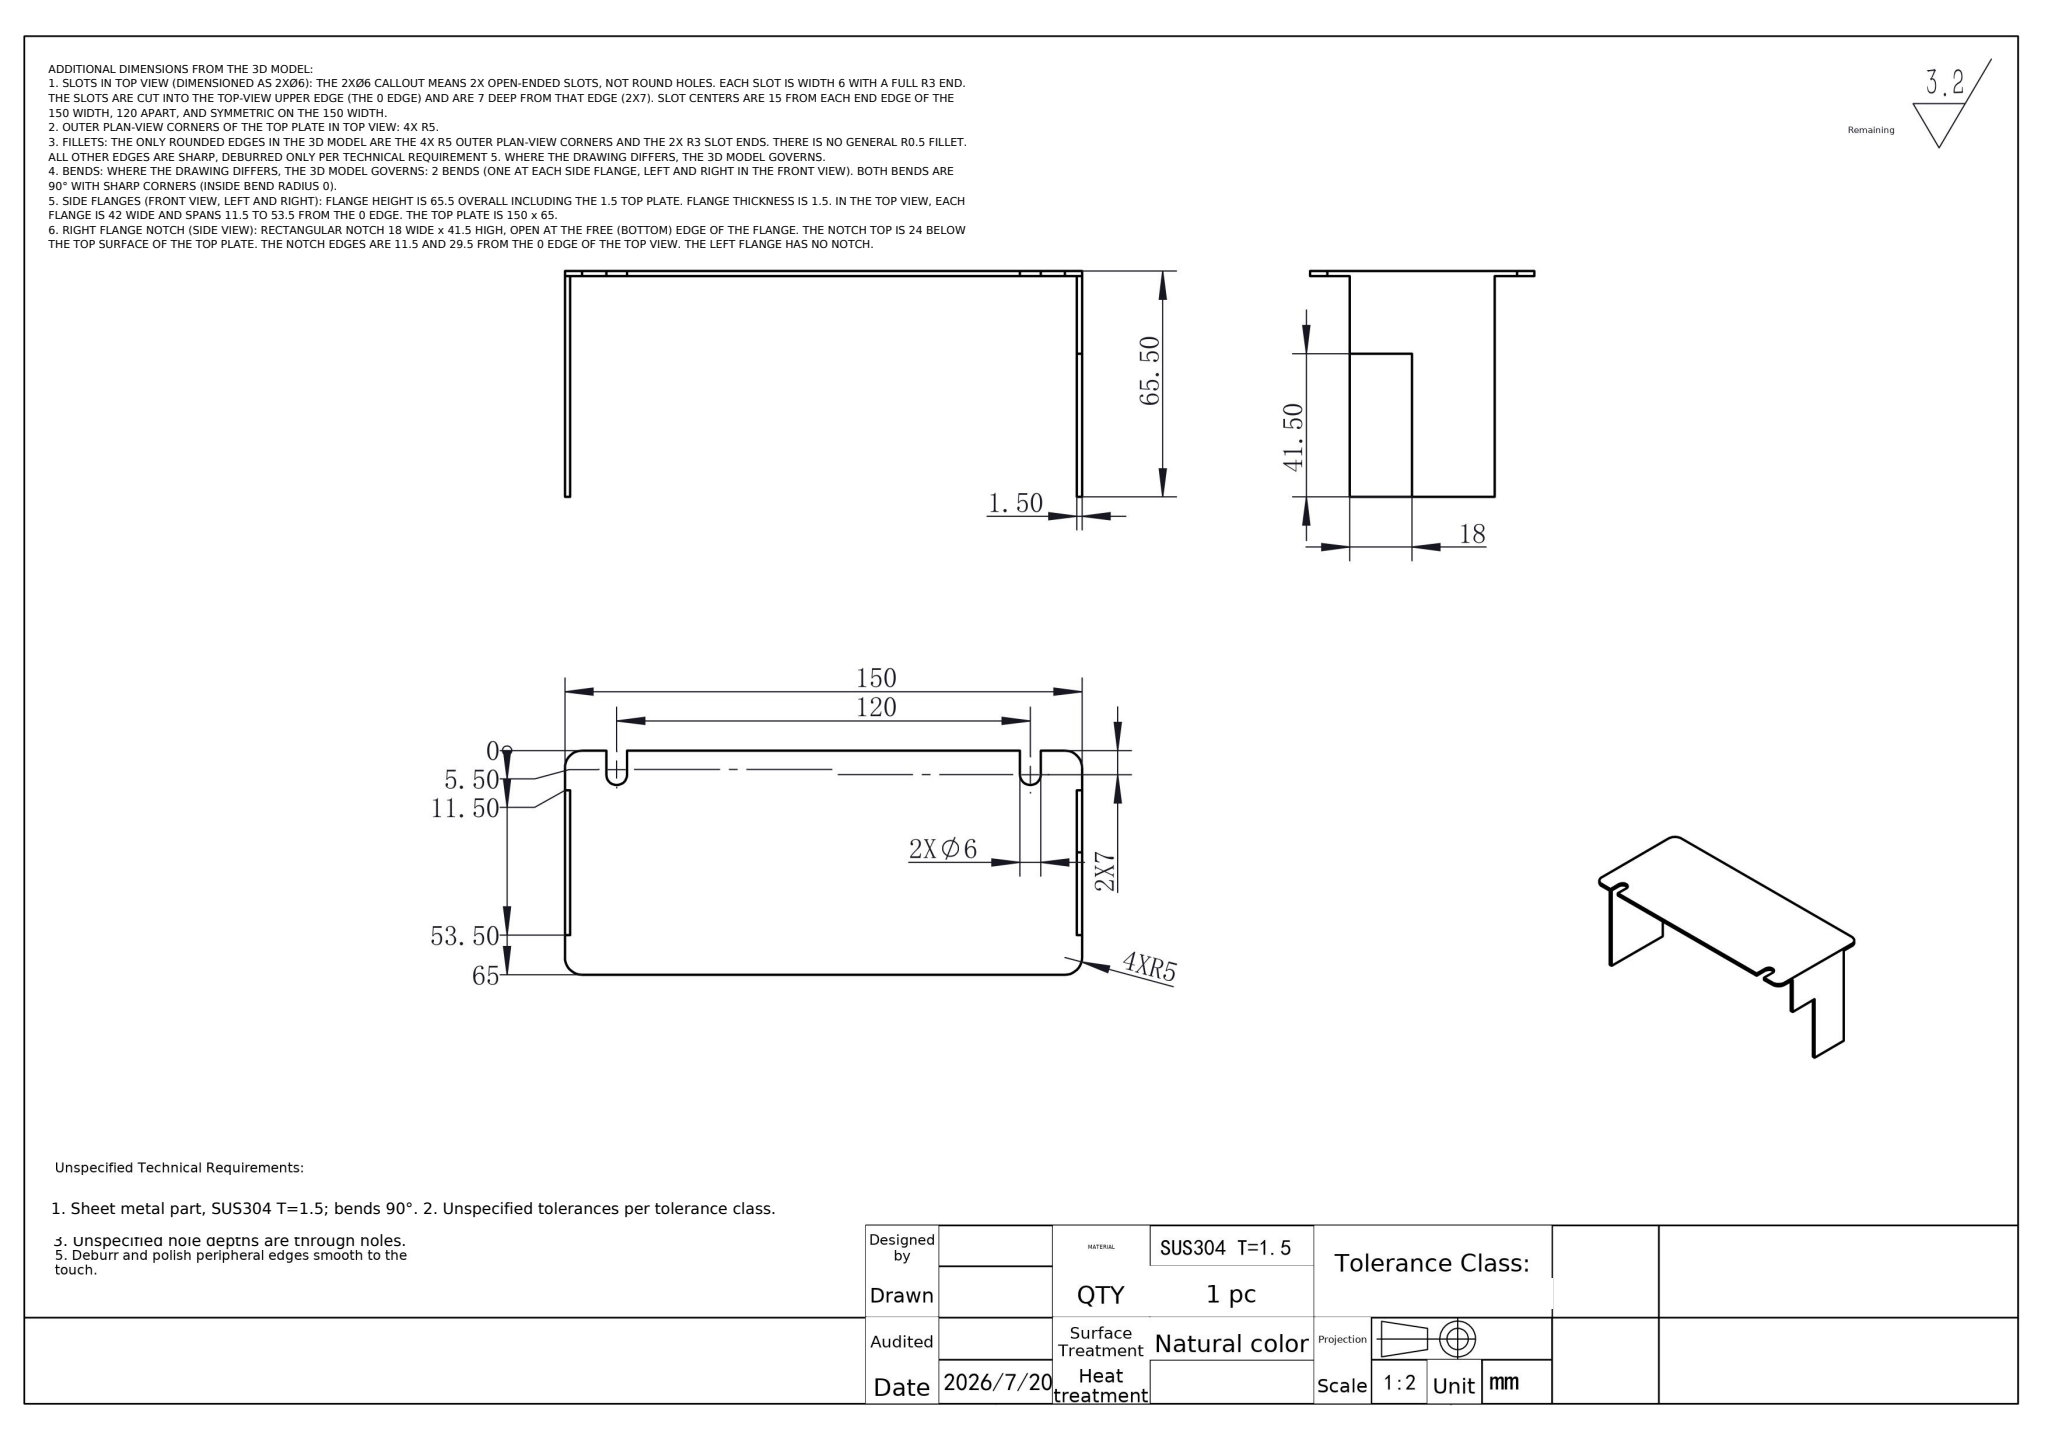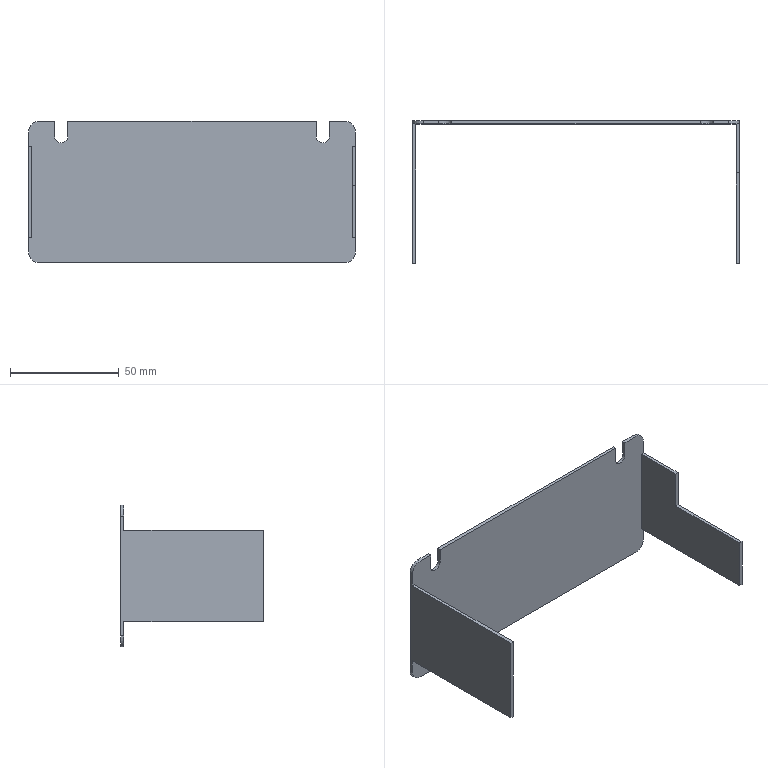Part | NX | mm | 1 solid | 28 faces | box 150 x 65.5 x 65 mm | volume 21368 mm3 | plane 22 | cylinder 6 | commonest cylinder face diameters 10 x4 6 x2
STEP:
#1=CARTESIAN_POINT('',(75.,0.,27.5));
#2=VERTEX_POINT('',#1);
#3=CARTESIAN_POINT('',(75.,0.,-27.5));
#4=VERTEX_POINT('',#3);
#5=CARTESIAN_POINT('',(75.,0.,32.5));
#6=DIRECTION('',(0.,0.,-1.));
#7=VECTOR('',#6,1000.);
#8=LINE('',#5,#7);
#9=EDGE_CURVE('',#2,#4,#8,.T.);
#10=ORIENTED_EDGE('',*,*,#9,.F.);
#11=CARTESIAN_POINT('',(75.,-1.5,27.5));
#12=VERTEX_POINT('',#11);
#13=CARTESIAN_POINT('',(75.,-1.5,27.5));
#14=DIRECTION('',(0.,-1.,0.));
#15=VECTOR('',#14,1000.);
#16=LINE('',#13,#15);
#17=EDGE_CURVE('',#2,#12,#16,.T.);
#18=ORIENTED_EDGE('',*,*,#17,.T.);
#19=CARTESIAN_POINT('',(75.,-1.5,21.));
#20=VERTEX_POINT('',#19);
#21=CARTESIAN_POINT('',(75.,-1.5,32.5));
#22=DIRECTION('',(0.,0.,-1.));
#23=VECTOR('',#22,1000.);
#24=LINE('',#21,#23);
#25=EDGE_CURVE('',#12,#20,#24,.T.);
#26=ORIENTED_EDGE('',*,*,#25,.T.);
#27=CARTESIAN_POINT('',(75.,-24.,21.));
#28=VERTEX_POINT('',#27);
#29=CARTESIAN_POINT('',(75.,-65.5,21.));
#30=DIRECTION('',(0.,1.,0.));
#31=VECTOR('',#30,1000.);
#32=LINE('',#29,#31);
#33=EDGE_CURVE('',#28,#20,#32,.T.);
#34=ORIENTED_EDGE('',*,*,#33,.F.);
#35=CARTESIAN_POINT('',(75.,-24.,3.));
#36=VERTEX_POINT('',#35);
#37=CARTESIAN_POINT('',(75.,-24.,3.));
#38=DIRECTION('',(0.,0.,-1.));
#39=VECTOR('',#38,1000.);
#40=LINE('',#37,#39);
#41=EDGE_CURVE('',#28,#36,#40,.T.);
#42=ORIENTED_EDGE('',*,*,#41,.T.);
#43=CARTESIAN_POINT('',(75.,-65.5,3.));
#44=VERTEX_POINT('',#43);
#45=CARTESIAN_POINT('',(75.,-100.5,3.));
#46=DIRECTION('',(0.,-1.,0.));
#47=VECTOR('',#46,1000.);
#48=LINE('',#45,#47);
#49=EDGE_CURVE('',#36,#44,#48,.T.);
#50=ORIENTED_EDGE('',*,*,#49,.T.);
#51=CARTESIAN_POINT('',(75.,-65.5,-21.));
#52=VERTEX_POINT('',#51);
#53=CARTESIAN_POINT('',(75.,-65.5,21.));
#54=DIRECTION('',(0.,0.,1.));
#55=VECTOR('',#54,1000.);
#56=LINE('',#53,#55);
#57=EDGE_CURVE('',#52,#44,#56,.T.);
#58=ORIENTED_EDGE('',*,*,#57,.F.);
#59=CARTESIAN_POINT('',(75.,-1.5,-21.));
#60=VERTEX_POINT('',#59);
#61=CARTESIAN_POINT('',(75.,-65.5,-21.));
#62=DIRECTION('',(0.,1.,0.));
#63=VECTOR('',#62,1000.);
#64=LINE('',#61,#63);
#65=EDGE_CURVE('',#52,#60,#64,.T.);
#66=ORIENTED_EDGE('',*,*,#65,.T.);
#67=CARTESIAN_POINT('',(75.,-1.5,-27.5));
#68=VERTEX_POINT('',#67);
#69=CARTESIAN_POINT('',(75.,-1.5,32.5));
#70=DIRECTION('',(0.,0.,-1.));
#71=VECTOR('',#70,1000.);
#72=LINE('',#69,#71);
#73=EDGE_CURVE('',#60,#68,#72,.T.);
#74=ORIENTED_EDGE('',*,*,#73,.T.);
#75=CARTESIAN_POINT('',(75.,-1.5,-27.5));
#76=DIRECTION('',(0.,1.,0.));
#77=VECTOR('',#76,1000.);
#78=LINE('',#75,#77);
#79=EDGE_CURVE('',#68,#4,#78,.T.);
#80=ORIENTED_EDGE('',*,*,#79,.T.);
#81=EDGE_LOOP('',(#10,#18,#26,#34,#42,#50,#58,#66,#74,#80));
#82=FACE_OUTER_BOUND('',#81,.T.);
#83=CARTESIAN_POINT('',(75.,-1.5,32.5));
#84=DIRECTION('',(1.,0.,0.));
#85=DIRECTION('',(0.,0.,-1.));
#86=AXIS2_PLACEMENT_3D('',#83,#84,#85);
#87=PLANE('',#86);
#88=ADVANCED_FACE('',(#82),#87,.T.);
#89=CARTESIAN_POINT('',(73.5,-24.,21.));
#90=VERTEX_POINT('',#89);
#91=CARTESIAN_POINT('',(73.,-24.,21.));
#92=DIRECTION('',(1.,0.,0.));
#93=VECTOR('',#92,1000.);
#94=LINE('',#91,#93);
#95=EDGE_CURVE('',#90,#28,#94,.T.);
#96=ORIENTED_EDGE('',*,*,#95,.T.);
#97=ORIENTED_EDGE('',*,*,#33,.T.);
#98=CARTESIAN_POINT('',(73.5,-1.5,21.));
#99=VERTEX_POINT('',#98);
#100=CARTESIAN_POINT('',(75.,-1.5,21.));
#101=DIRECTION('',(-1.,0.,0.));
#102=VECTOR('',#101,1000.);
#103=LINE('',#100,#102);
#104=EDGE_CURVE('',#20,#99,#103,.T.);
#105=ORIENTED_EDGE('',*,*,#104,.T.);
#106=CARTESIAN_POINT('',(73.5,-65.5,21.));
#107=DIRECTION('',(0.,1.,0.));
#108=VECTOR('',#107,1000.);
#109=LINE('',#106,#108);
#110=EDGE_CURVE('',#90,#99,#109,.T.);
#111=ORIENTED_EDGE('',*,*,#110,.F.);
#112=EDGE_LOOP('',(#96,#97,#105,#111));
#113=FACE_OUTER_BOUND('',#112,.T.);
#114=CARTESIAN_POINT('',(75.,-65.5,21.));
#115=DIRECTION('',(-0.,0.,-1.));
#116=DIRECTION('',(-1.,0.,0.));
#117=AXIS2_PLACEMENT_3D('',#114,#115,#116);
#118=PLANE('',#117);
#119=ADVANCED_FACE('',(#113),#118,.F.);
#120=CARTESIAN_POINT('',(73.5,-24.,3.));
#121=VERTEX_POINT('',#120);
#122=CARTESIAN_POINT('',(73.5,-65.5,3.));
#123=VERTEX_POINT('',#122);
#124=CARTESIAN_POINT('',(73.5,-65.5,3.));
#125=DIRECTION('',(0.,-1.,0.));
#126=VECTOR('',#125,1000.);
#127=LINE('',#124,#126);
#128=EDGE_CURVE('',#121,#123,#127,.T.);
#129=ORIENTED_EDGE('',*,*,#128,.F.);
#130=CARTESIAN_POINT('',(73.5,-24.,21.));
#131=DIRECTION('',(0.,0.,-1.));
#132=VECTOR('',#131,1000.);
#133=LINE('',#130,#132);
#134=EDGE_CURVE('',#90,#121,#133,.T.);
#135=ORIENTED_EDGE('',*,*,#134,.F.);
#136=ORIENTED_EDGE('',*,*,#110,.T.);
#137=CARTESIAN_POINT('',(73.5,-1.5,-21.));
#138=VERTEX_POINT('',#137);
#139=CARTESIAN_POINT('',(73.5,-1.5,21.));
#140=DIRECTION('',(0.,0.,-1.));
#141=VECTOR('',#140,1000.);
#142=LINE('',#139,#141);
#143=EDGE_CURVE('',#99,#138,#142,.T.);
#144=ORIENTED_EDGE('',*,*,#143,.T.);
#145=CARTESIAN_POINT('',(73.5,-65.5,-21.));
#146=VERTEX_POINT('',#145);
#147=CARTESIAN_POINT('',(73.5,-65.5,-21.));
#148=DIRECTION('',(0.,1.,0.));
#149=VECTOR('',#148,1000.);
#150=LINE('',#147,#149);
#151=EDGE_CURVE('',#146,#138,#150,.T.);
#152=ORIENTED_EDGE('',*,*,#151,.F.);
#153=CARTESIAN_POINT('',(73.5,-65.5,21.));
#154=DIRECTION('',(0.,0.,-1.));
#155=VECTOR('',#154,1000.);
#156=LINE('',#153,#155);
#157=EDGE_CURVE('',#123,#146,#156,.T.);
#158=ORIENTED_EDGE('',*,*,#157,.F.);
#159=EDGE_LOOP('',(#129,#135,#136,#144,#152,#158));
#160=FACE_OUTER_BOUND('',#159,.T.);
#161=CARTESIAN_POINT('',(73.5,-65.5,21.));
#162=DIRECTION('',(1.,0.,0.));
#163=DIRECTION('',(0.,0.,-1.));
#164=AXIS2_PLACEMENT_3D('',#161,#162,#163);
#165=PLANE('',#164);
#166=ADVANCED_FACE('',(#160),#165,.F.);
#167=CARTESIAN_POINT('',(0.,-65.5,3.));
#168=DIRECTION('',(1.,0.,0.));
#169=VECTOR('',#168,1000.);
#170=LINE('',#167,#169);
#171=EDGE_CURVE('',#123,#44,#170,.T.);
#172=ORIENTED_EDGE('',*,*,#171,.F.);
#173=ORIENTED_EDGE('',*,*,#157,.T.);
#174=CARTESIAN_POINT('',(75.,-65.5,-21.));
#175=DIRECTION('',(1.,0.,0.));
#176=VECTOR('',#175,1000.);
#177=LINE('',#174,#176);
#178=EDGE_CURVE('',#146,#52,#177,.T.);
#179=ORIENTED_EDGE('',*,*,#178,.T.);
#180=ORIENTED_EDGE('',*,*,#57,.T.);
#181=EDGE_LOOP('',(#172,#173,#179,#180));
#182=FACE_OUTER_BOUND('',#181,.T.);
#183=CARTESIAN_POINT('',(0.,-65.5,0.));
#184=DIRECTION('',(0.,1.,0.));
#185=DIRECTION('',(0.,0.,1.));
#186=AXIS2_PLACEMENT_3D('',#183,#184,#185);
#187=PLANE('',#186);
#188=ADVANCED_FACE('',(#182),#187,.F.);
#189=CARTESIAN_POINT('',(57.,-1.5,32.5));
#190=VERTEX_POINT('',#189);
#191=CARTESIAN_POINT('',(57.,0.,32.5));
#192=VERTEX_POINT('',#191);
#193=CARTESIAN_POINT('',(57.,-2.,32.5));
#194=DIRECTION('',(0.,1.,0.));
#195=VECTOR('',#194,1000.);
#196=LINE('',#193,#195);
#197=EDGE_CURVE('',#190,#192,#196,.T.);
#198=ORIENTED_EDGE('',*,*,#197,.T.);
#199=CARTESIAN_POINT('',(-57.,0.,32.5));
#200=VERTEX_POINT('',#199);
#201=CARTESIAN_POINT('',(-75.,0.,32.5));
#202=DIRECTION('',(1.,0.,0.));
#203=VECTOR('',#202,1000.);
#204=LINE('',#201,#203);
#205=EDGE_CURVE('',#200,#192,#204,.T.);
#206=ORIENTED_EDGE('',*,*,#205,.F.);
#207=CARTESIAN_POINT('',(-57.,-1.5,32.5));
#208=VERTEX_POINT('',#207);
#209=CARTESIAN_POINT('',(-57.,-2.,32.5));
#210=DIRECTION('',(0.,1.,0.));
#211=VECTOR('',#210,1000.);
#212=LINE('',#209,#211);
#213=EDGE_CURVE('',#208,#200,#212,.T.);
#214=ORIENTED_EDGE('',*,*,#213,.F.);
#215=CARTESIAN_POINT('',(-75.,-1.5,32.5));
#216=DIRECTION('',(1.,0.,0.));
#217=VECTOR('',#216,1000.);
#218=LINE('',#215,#217);
#219=EDGE_CURVE('',#208,#190,#218,.T.);
#220=ORIENTED_EDGE('',*,*,#219,.T.);
#221=EDGE_LOOP('',(#198,#206,#214,#220));
#222=FACE_OUTER_BOUND('',#221,.T.);
#223=CARTESIAN_POINT('',(-75.,-1.5,32.5));
#224=DIRECTION('',(0.,0.,1.));
#225=DIRECTION('',(1.,0.,0.));
#226=AXIS2_PLACEMENT_3D('',#223,#224,#225);
#227=PLANE('',#226);
#228=ADVANCED_FACE('',(#222),#227,.T.);
#229=CARTESIAN_POINT('',(-70.,0.,32.5));
#230=VERTEX_POINT('',#229);
#231=CARTESIAN_POINT('',(-63.,0.,32.5));
#232=VERTEX_POINT('',#231);
#233=CARTESIAN_POINT('',(-75.,0.,32.5));
#234=DIRECTION('',(1.,0.,0.));
#235=VECTOR('',#234,1000.);
#236=LINE('',#233,#235);
#237=EDGE_CURVE('',#230,#232,#236,.T.);
#238=ORIENTED_EDGE('',*,*,#237,.F.);
#239=CARTESIAN_POINT('',(-70.,-1.5,32.5));
#240=VERTEX_POINT('',#239);
#241=CARTESIAN_POINT('',(-70.,-1.5,32.5));
#242=DIRECTION('',(0.,-1.,0.));
#243=VECTOR('',#242,1000.);
#244=LINE('',#241,#243);
#245=EDGE_CURVE('',#230,#240,#244,.T.);
#246=ORIENTED_EDGE('',*,*,#245,.T.);
#247=CARTESIAN_POINT('',(-63.,-1.5,32.5));
#248=VERTEX_POINT('',#247);
#249=CARTESIAN_POINT('',(-75.,-1.5,32.5));
#250=DIRECTION('',(1.,0.,0.));
#251=VECTOR('',#250,1000.);
#252=LINE('',#249,#251);
#253=EDGE_CURVE('',#240,#248,#252,.T.);
#254=ORIENTED_EDGE('',*,*,#253,.T.);
#255=CARTESIAN_POINT('',(-63.,-2.,32.5));
#256=DIRECTION('',(0.,1.,0.));
#257=VECTOR('',#256,1000.);
#258=LINE('',#255,#257);
#259=EDGE_CURVE('',#248,#232,#258,.T.);
#260=ORIENTED_EDGE('',*,*,#259,.T.);
#261=EDGE_LOOP('',(#238,#246,#254,#260));
#262=FACE_OUTER_BOUND('',#261,.T.);
#263=CARTESIAN_POINT('',(-75.,-1.5,32.5));
#264=DIRECTION('',(0.,0.,1.));
#265=DIRECTION('',(1.,0.,0.));
#266=AXIS2_PLACEMENT_3D('',#263,#264,#265);
#267=PLANE('',#266);
#268=ADVANCED_FACE('',(#262),#267,.T.);
#269=ORIENTED_EDGE('',*,*,#25,.F.);
#270=CARTESIAN_POINT('',(70.,-1.5,32.5));
#271=VERTEX_POINT('',#270);
#272=CARTESIAN_POINT('',(70.,-1.5,27.5));
#273=DIRECTION('',(0.,-1.,0.));
#274=DIRECTION('',(0.,0.,-1.));
#275=AXIS2_PLACEMENT_3D('',#272,#273,#274);
#276=CIRCLE('',#275,5.);
#277=EDGE_CURVE('',#12,#271,#276,.T.);
#278=ORIENTED_EDGE('',*,*,#277,.T.);
#279=CARTESIAN_POINT('',(63.,-1.5,32.5));
#280=VERTEX_POINT('',#279);
#281=CARTESIAN_POINT('',(-75.,-1.5,32.5));
#282=DIRECTION('',(1.,0.,0.));
#283=VECTOR('',#282,1000.);
#284=LINE('',#281,#283);
#285=EDGE_CURVE('',#280,#271,#284,.T.);
#286=ORIENTED_EDGE('',*,*,#285,.F.);
#287=CARTESIAN_POINT('',(63.,-1.5,25.5));
#288=VERTEX_POINT('',#287);
#289=CARTESIAN_POINT('',(63.,-1.5,0.));
#290=DIRECTION('',(0.,0.,1.));
#291=VECTOR('',#290,1000.);
#292=LINE('',#289,#291);
#293=EDGE_CURVE('',#288,#280,#292,.T.);
#294=ORIENTED_EDGE('',*,*,#293,.F.);
#295=CARTESIAN_POINT('',(57.,-1.5,25.5));
#296=VERTEX_POINT('',#295);
#297=CARTESIAN_POINT('',(60.,-1.5,25.5));
#298=DIRECTION('',(0.,-1.,0.));
#299=DIRECTION('',(0.,0.,-1.));
#300=AXIS2_PLACEMENT_3D('',#297,#298,#299);
#301=CIRCLE('',#300,3.);
#302=EDGE_CURVE('',#296,#288,#301,.T.);
#303=ORIENTED_EDGE('',*,*,#302,.F.);
#304=CARTESIAN_POINT('',(57.,-1.5,0.));
#305=DIRECTION('',(0.,0.,-1.));
#306=VECTOR('',#305,1000.);
#307=LINE('',#304,#306);
#308=EDGE_CURVE('',#190,#296,#307,.T.);
#309=ORIENTED_EDGE('',*,*,#308,.F.);
#310=ORIENTED_EDGE('',*,*,#219,.F.);
#311=CARTESIAN_POINT('',(-57.,-1.5,25.5));
#312=VERTEX_POINT('',#311);
#313=CARTESIAN_POINT('',(-57.,-1.5,0.));
#314=DIRECTION('',(0.,0.,1.));
#315=VECTOR('',#314,1000.);
#316=LINE('',#313,#315);
#317=EDGE_CURVE('',#312,#208,#316,.T.);
#318=ORIENTED_EDGE('',*,*,#317,.F.);
#319=CARTESIAN_POINT('',(-63.,-1.5,25.5));
#320=VERTEX_POINT('',#319);
#321=CARTESIAN_POINT('',(-60.,-1.5,25.5));
#322=DIRECTION('',(0.,-1.,0.));
#323=DIRECTION('',(0.,0.,-1.));
#324=AXIS2_PLACEMENT_3D('',#321,#322,#323);
#325=CIRCLE('',#324,3.);
#326=EDGE_CURVE('',#320,#312,#325,.T.);
#327=ORIENTED_EDGE('',*,*,#326,.F.);
#328=CARTESIAN_POINT('',(-63.,-1.5,0.));
#329=DIRECTION('',(0.,0.,-1.));
#330=VECTOR('',#329,1000.);
#331=LINE('',#328,#330);
#332=EDGE_CURVE('',#248,#320,#331,.T.);
#333=ORIENTED_EDGE('',*,*,#332,.F.);
#334=ORIENTED_EDGE('',*,*,#253,.F.);
#335=CARTESIAN_POINT('',(-75.,-1.5,27.5));
#336=VERTEX_POINT('',#335);
#337=CARTESIAN_POINT('',(-70.,-1.5,27.5));
#338=DIRECTION('',(0.,-1.,0.));
#339=DIRECTION('',(0.,0.,-1.));
#340=AXIS2_PLACEMENT_3D('',#337,#338,#339);
#341=CIRCLE('',#340,5.);
#342=EDGE_CURVE('',#240,#336,#341,.T.);
#343=ORIENTED_EDGE('',*,*,#342,.T.);
#344=CARTESIAN_POINT('',(-75.,-1.5,21.));
#345=VERTEX_POINT('',#344);
#346=CARTESIAN_POINT('',(-75.,-1.5,32.5));
#347=DIRECTION('',(0.,0.,1.));
#348=VECTOR('',#347,1000.);
#349=LINE('',#346,#348);
#350=EDGE_CURVE('',#345,#336,#349,.T.);
#351=ORIENTED_EDGE('',*,*,#350,.F.);
#352=CARTESIAN_POINT('',(-73.5,-1.5,21.));
#353=VERTEX_POINT('',#352);
#354=CARTESIAN_POINT('',(-75.,-1.5,21.));
#355=DIRECTION('',(-1.,0.,0.));
#356=VECTOR('',#355,1000.);
#357=LINE('',#354,#356);
#358=EDGE_CURVE('',#353,#345,#357,.T.);
#359=ORIENTED_EDGE('',*,*,#358,.F.);
#360=CARTESIAN_POINT('',(-73.5,-1.5,-21.));
#361=VERTEX_POINT('',#360);
#362=CARTESIAN_POINT('',(-73.5,-1.5,21.));
#363=DIRECTION('',(0.,0.,1.));
#364=VECTOR('',#363,1000.);
#365=LINE('',#362,#364);
#366=EDGE_CURVE('',#361,#353,#365,.T.);
#367=ORIENTED_EDGE('',*,*,#366,.F.);
#368=CARTESIAN_POINT('',(-75.,-1.5,-21.));
#369=VERTEX_POINT('',#368);
#370=CARTESIAN_POINT('',(-75.,-1.5,-21.));
#371=DIRECTION('',(1.,0.,0.));
#372=VECTOR('',#371,1000.);
#373=LINE('',#370,#372);
#374=EDGE_CURVE('',#369,#361,#373,.T.);
#375=ORIENTED_EDGE('',*,*,#374,.F.);
#376=CARTESIAN_POINT('',(-75.,-1.5,-27.5));
#377=VERTEX_POINT('',#376);
#378=CARTESIAN_POINT('',(-75.,-1.5,32.5));
#379=DIRECTION('',(0.,0.,1.));
#380=VECTOR('',#379,1000.);
#381=LINE('',#378,#380);
#382=EDGE_CURVE('',#377,#369,#381,.T.);
#383=ORIENTED_EDGE('',*,*,#382,.F.);
#384=CARTESIAN_POINT('',(-70.,-1.5,-32.5));
#385=VERTEX_POINT('',#384);
#386=CARTESIAN_POINT('',(-70.,-1.5,-27.5));
#387=DIRECTION('',(0.,-1.,0.));
#388=DIRECTION('',(0.,0.,-1.));
#389=AXIS2_PLACEMENT_3D('',#386,#387,#388);
#390=CIRCLE('',#389,5.);
#391=EDGE_CURVE('',#377,#385,#390,.T.);
#392=ORIENTED_EDGE('',*,*,#391,.T.);
#393=CARTESIAN_POINT('',(70.,-1.5,-32.5));
#394=VERTEX_POINT('',#393);
#395=CARTESIAN_POINT('',(-75.,-1.5,-32.5));
#396=DIRECTION('',(-1.,0.,0.));
#397=VECTOR('',#396,1000.);
#398=LINE('',#395,#397);
#399=EDGE_CURVE('',#394,#385,#398,.T.);
#400=ORIENTED_EDGE('',*,*,#399,.F.);
#401=CARTESIAN_POINT('',(70.,-1.5,-27.5));
#402=DIRECTION('',(0.,-1.,0.));
#403=DIRECTION('',(0.,0.,-1.));
#404=AXIS2_PLACEMENT_3D('',#401,#402,#403);
#405=CIRCLE('',#404,5.);
#406=EDGE_CURVE('',#394,#68,#405,.T.);
#407=ORIENTED_EDGE('',*,*,#406,.T.);
#408=ORIENTED_EDGE('',*,*,#73,.F.);
#409=CARTESIAN_POINT('',(75.,-1.5,-21.));
#410=DIRECTION('',(1.,0.,0.));
#411=VECTOR('',#410,1000.);
#412=LINE('',#409,#411);
#413=EDGE_CURVE('',#138,#60,#412,.T.);
#414=ORIENTED_EDGE('',*,*,#413,.F.);
#415=ORIENTED_EDGE('',*,*,#143,.F.);
#416=ORIENTED_EDGE('',*,*,#104,.F.);
#417=EDGE_LOOP('',(#269,#278,#286,#294,#303,#309,#310,#318,#327,#333,#334,#343,#351,#359,#367,#375,#383,#392,#400,#407,#408,#414,#415,#416));
#418=FACE_OUTER_BOUND('',#417,.T.);
#419=CARTESIAN_POINT('',(0.,-1.5,0.));
#420=DIRECTION('',(0.,-1.,0.));
#421=DIRECTION('',(0.,0.,-1.));
#422=AXIS2_PLACEMENT_3D('',#419,#420,#421);
#423=PLANE('',#422);
#424=ADVANCED_FACE('',(#418),#423,.T.);
#425=ORIENTED_EDGE('',*,*,#285,.T.);
#426=CARTESIAN_POINT('',(70.,0.,32.5));
#427=VERTEX_POINT('',#426);
#428=CARTESIAN_POINT('',(70.,-1.5,32.5));
#429=DIRECTION('',(0.,1.,0.));
#430=VECTOR('',#429,1000.);
#431=LINE('',#428,#430);
#432=EDGE_CURVE('',#271,#427,#431,.T.);
#433=ORIENTED_EDGE('',*,*,#432,.T.);
#434=CARTESIAN_POINT('',(63.,0.,32.5));
#435=VERTEX_POINT('',#434);
#436=CARTESIAN_POINT('',(-75.,0.,32.5));
#437=DIRECTION('',(1.,0.,0.));
#438=VECTOR('',#437,1000.);
#439=LINE('',#436,#438);
#440=EDGE_CURVE('',#435,#427,#439,.T.);
#441=ORIENTED_EDGE('',*,*,#440,.F.);
#442=CARTESIAN_POINT('',(63.,-2.,32.5));
#443=DIRECTION('',(0.,1.,0.));
#444=VECTOR('',#443,1000.);
#445=LINE('',#442,#444);
#446=EDGE_CURVE('',#280,#435,#445,.T.);
#447=ORIENTED_EDGE('',*,*,#446,.F.);
#448=EDGE_LOOP('',(#425,#433,#441,#447));
#449=FACE_OUTER_BOUND('',#448,.T.);
#450=CARTESIAN_POINT('',(-75.,-1.5,32.5));
#451=DIRECTION('',(0.,0.,1.));
#452=DIRECTION('',(1.,0.,0.));
#453=AXIS2_PLACEMENT_3D('',#450,#451,#452);
#454=PLANE('',#453);
#455=ADVANCED_FACE('',(#449),#454,.T.);
#456=ORIENTED_EDGE('',*,*,#350,.T.);
#457=CARTESIAN_POINT('',(-75.,0.,27.5));
#458=VERTEX_POINT('',#457);
#459=CARTESIAN_POINT('',(-75.,-1.5,27.5));
#460=DIRECTION('',(0.,1.,0.));
#461=VECTOR('',#460,1000.);
#462=LINE('',#459,#461);
#463=EDGE_CURVE('',#336,#458,#462,.T.);
#464=ORIENTED_EDGE('',*,*,#463,.T.);
#465=CARTESIAN_POINT('',(-75.,0.,-27.5));
#466=VERTEX_POINT('',#465);
#467=CARTESIAN_POINT('',(-75.,0.,32.5));
#468=DIRECTION('',(0.,0.,1.));
#469=VECTOR('',#468,1000.);
#470=LINE('',#467,#469);
#471=EDGE_CURVE('',#466,#458,#470,.T.);
#472=ORIENTED_EDGE('',*,*,#471,.F.);
#473=CARTESIAN_POINT('',(-75.,-1.5,-27.5));
#474=DIRECTION('',(0.,-1.,0.));
#475=VECTOR('',#474,1000.);
#476=LINE('',#473,#475);
#477=EDGE_CURVE('',#466,#377,#476,.T.);
#478=ORIENTED_EDGE('',*,*,#477,.T.);
#479=ORIENTED_EDGE('',*,*,#382,.T.);
#480=CARTESIAN_POINT('',(-75.,-65.5,-21.));
#481=VERTEX_POINT('',#480);
#482=CARTESIAN_POINT('',(-75.,-65.5,-21.));
#483=DIRECTION('',(0.,1.,0.));
#484=VECTOR('',#483,1000.);
#485=LINE('',#482,#484);
#486=EDGE_CURVE('',#481,#369,#485,.T.);
#487=ORIENTED_EDGE('',*,*,#486,.F.);
#488=CARTESIAN_POINT('',(-75.,-65.5,21.));
#489=VERTEX_POINT('',#488);
#490=CARTESIAN_POINT('',(-75.,-65.5,21.));
#491=DIRECTION('',(0.,0.,-1.));
#492=VECTOR('',#491,1000.);
#493=LINE('',#490,#492);
#494=EDGE_CURVE('',#489,#481,#493,.T.);
#495=ORIENTED_EDGE('',*,*,#494,.F.);
#496=CARTESIAN_POINT('',(-75.,-65.5,21.));
#497=DIRECTION('',(0.,1.,0.));
#498=VECTOR('',#497,1000.);
#499=LINE('',#496,#498);
#500=EDGE_CURVE('',#489,#345,#499,.T.);
#501=ORIENTED_EDGE('',*,*,#500,.T.);
#502=EDGE_LOOP('',(#456,#464,#472,#478,#479,#487,#495,#501));
#503=FACE_OUTER_BOUND('',#502,.T.);
#504=CARTESIAN_POINT('',(-75.,-1.5,32.5));
#505=DIRECTION('',(-1.,0.,0.));
#506=DIRECTION('',(0.,0.,1.));
#507=AXIS2_PLACEMENT_3D('',#504,#505,#506);
#508=PLANE('',#507);
#509=ADVANCED_FACE('',(#503),#508,.T.);
#510=ORIENTED_EDGE('',*,*,#399,.T.);
#511=CARTESIAN_POINT('',(-70.,0.,-32.5));
#512=VERTEX_POINT('',#511);
#513=CARTESIAN_POINT('',(-70.,-1.5,-32.5));
#514=DIRECTION('',(0.,1.,0.));
#515=VECTOR('',#514,1000.);
#516=LINE('',#513,#515);
#517=EDGE_CURVE('',#385,#512,#516,.T.);
#518=ORIENTED_EDGE('',*,*,#517,.T.);
#519=CARTESIAN_POINT('',(70.,0.,-32.5));
#520=VERTEX_POINT('',#519);
#521=CARTESIAN_POINT('',(-75.,0.,-32.5));
#522=DIRECTION('',(-1.,0.,0.));
#523=VECTOR('',#522,1000.);
#524=LINE('',#521,#523);
#525=EDGE_CURVE('',#520,#512,#524,.T.);
#526=ORIENTED_EDGE('',*,*,#525,.F.);
#527=CARTESIAN_POINT('',(70.,-1.5,-32.5));
#528=DIRECTION('',(0.,-1.,0.));
#529=VECTOR('',#528,1000.);
#530=LINE('',#527,#529);
#531=EDGE_CURVE('',#520,#394,#530,.T.);
#532=ORIENTED_EDGE('',*,*,#531,.T.);
#533=EDGE_LOOP('',(#510,#518,#526,#532));
#534=FACE_OUTER_BOUND('',#533,.T.);
#535=CARTESIAN_POINT('',(-75.,-1.5,-32.5));
#536=DIRECTION('',(0.,0.,-1.));
#537=DIRECTION('',(-1.,0.,0.));
#538=AXIS2_PLACEMENT_3D('',#535,#536,#537);
#539=PLANE('',#538);
#540=ADVANCED_FACE('',(#534),#539,.T.);
#541=ORIENTED_EDGE('',*,*,#440,.T.);
#542=CARTESIAN_POINT('',(70.,0.,27.5));
#543=DIRECTION('',(0.,1.,0.));
#544=DIRECTION('',(0.,0.,-1.));
#545=AXIS2_PLACEMENT_3D('',#542,#543,#544);
#546=CIRCLE('',#545,5.);
#547=EDGE_CURVE('',#427,#2,#546,.T.);
#548=ORIENTED_EDGE('',*,*,#547,.T.);
#549=ORIENTED_EDGE('',*,*,#9,.T.);
#550=CARTESIAN_POINT('',(70.,0.,-27.5));
#551=DIRECTION('',(0.,1.,0.));
#552=DIRECTION('',(0.,0.,-1.));
#553=AXIS2_PLACEMENT_3D('',#550,#551,#552);
#554=CIRCLE('',#553,5.);
#555=EDGE_CURVE('',#4,#520,#554,.T.);
#556=ORIENTED_EDGE('',*,*,#555,.T.);
#557=ORIENTED_EDGE('',*,*,#525,.T.);
#558=CARTESIAN_POINT('',(-70.,0.,-27.5));
#559=DIRECTION('',(0.,1.,0.));
#560=DIRECTION('',(0.,0.,-1.));
#561=AXIS2_PLACEMENT_3D('',#558,#559,#560);
#562=CIRCLE('',#561,5.);
#563=EDGE_CURVE('',#512,#466,#562,.T.);
#564=ORIENTED_EDGE('',*,*,#563,.T.);
#565=ORIENTED_EDGE('',*,*,#471,.T.);
#566=CARTESIAN_POINT('',(-70.,0.,27.5));
#567=DIRECTION('',(0.,1.,0.));
#568=DIRECTION('',(0.,0.,-1.));
#569=AXIS2_PLACEMENT_3D('',#566,#567,#568);
#570=CIRCLE('',#569,5.);
#571=EDGE_CURVE('',#458,#230,#570,.T.);
#572=ORIENTED_EDGE('',*,*,#571,.T.);
#573=ORIENTED_EDGE('',*,*,#237,.T.);
#574=CARTESIAN_POINT('',(-63.,0.,25.5));
#575=VERTEX_POINT('',#574);
#576=CARTESIAN_POINT('',(-63.,0.,32.5));
#577=DIRECTION('',(0.,0.,1.));
#578=VECTOR('',#577,1000.);
#579=LINE('',#576,#578);
#580=EDGE_CURVE('',#575,#232,#579,.T.);
#581=ORIENTED_EDGE('',*,*,#580,.F.);
#582=CARTESIAN_POINT('',(-57.,0.,25.5));
#583=VERTEX_POINT('',#582);
#584=CARTESIAN_POINT('',(-60.,0.,25.5));
#585=DIRECTION('',(0.,1.,0.));
#586=DIRECTION('',(0.,0.,1.));
#587=AXIS2_PLACEMENT_3D('',#584,#585,#586);
#588=CIRCLE('',#587,3.);
#589=EDGE_CURVE('',#583,#575,#588,.T.);
#590=ORIENTED_EDGE('',*,*,#589,.F.);
#591=CARTESIAN_POINT('',(-57.,0.,32.5));
#592=DIRECTION('',(0.,0.,-1.));
#593=VECTOR('',#592,1000.);
#594=LINE('',#591,#593);
#595=EDGE_CURVE('',#200,#583,#594,.T.);
#596=ORIENTED_EDGE('',*,*,#595,.F.);
#597=ORIENTED_EDGE('',*,*,#205,.T.);
#598=CARTESIAN_POINT('',(57.,0.,25.5));
#599=VERTEX_POINT('',#598);
#600=CARTESIAN_POINT('',(57.,0.,32.5));
#601=DIRECTION('',(-0.,0.,1.));
#602=VECTOR('',#601,1000.);
#603=LINE('',#600,#602);
#604=EDGE_CURVE('',#599,#192,#603,.T.);
#605=ORIENTED_EDGE('',*,*,#604,.F.);
#606=CARTESIAN_POINT('',(63.,0.,25.5));
#607=VERTEX_POINT('',#606);
#608=CARTESIAN_POINT('',(60.,0.,25.5));
#609=DIRECTION('',(0.,1.,0.));
#610=DIRECTION('',(0.,0.,1.));
#611=AXIS2_PLACEMENT_3D('',#608,#609,#610);
#612=CIRCLE('',#611,3.);
#613=EDGE_CURVE('',#607,#599,#612,.T.);
#614=ORIENTED_EDGE('',*,*,#613,.F.);
#615=CARTESIAN_POINT('',(63.,0.,32.5));
#616=DIRECTION('',(0.,0.,-1.));
#617=VECTOR('',#616,1000.);
#618=LINE('',#615,#617);
#619=EDGE_CURVE('',#435,#607,#618,.T.);
#620=ORIENTED_EDGE('',*,*,#619,.F.);
#621=EDGE_LOOP('',(#541,#548,#549,#556,#557,#564,#565,#572,#573,#581,#590,#596,#597,#605,#614,#620));
#622=FACE_OUTER_BOUND('',#621,.T.);
#623=CARTESIAN_POINT('',(0.,0.,0.));
#624=DIRECTION('',(0.,-1.,0.));
#625=DIRECTION('',(0.,0.,-1.));
#626=AXIS2_PLACEMENT_3D('',#623,#624,#625);
#627=PLANE('',#626);
#628=ADVANCED_FACE('',(#622),#627,.F.);
#629=ORIENTED_EDGE('',*,*,#413,.T.);
#630=ORIENTED_EDGE('',*,*,#65,.F.);
#631=ORIENTED_EDGE('',*,*,#178,.F.);
#632=ORIENTED_EDGE('',*,*,#151,.T.);
#633=EDGE_LOOP('',(#629,#630,#631,#632));
#634=FACE_OUTER_BOUND('',#633,.T.);
#635=CARTESIAN_POINT('',(75.,-65.5,-21.));
#636=DIRECTION('',(-0.,0.,1.));
#637=DIRECTION('',(1.,0.,0.));
#638=AXIS2_PLACEMENT_3D('',#635,#636,#637);
#639=PLANE('',#638);
#640=ADVANCED_FACE('',(#634),#639,.F.);
#641=ORIENTED_EDGE('',*,*,#374,.T.);
#642=CARTESIAN_POINT('',(-73.5,-65.5,-21.));
#643=VERTEX_POINT('',#642);
#644=CARTESIAN_POINT('',(-73.5,-65.5,-21.));
#645=DIRECTION('',(0.,1.,0.));
#646=VECTOR('',#645,1000.);
#647=LINE('',#644,#646);
#648=EDGE_CURVE('',#643,#361,#647,.T.);
#649=ORIENTED_EDGE('',*,*,#648,.F.);
#650=CARTESIAN_POINT('',(-75.,-65.5,-21.));
#651=DIRECTION('',(1.,0.,0.));
#652=VECTOR('',#651,1000.);
#653=LINE('',#650,#652);
#654=EDGE_CURVE('',#481,#643,#653,.T.);
#655=ORIENTED_EDGE('',*,*,#654,.F.);
#656=ORIENTED_EDGE('',*,*,#486,.T.);
#657=EDGE_LOOP('',(#641,#649,#655,#656));
#658=FACE_OUTER_BOUND('',#657,.T.);
#659=CARTESIAN_POINT('',(-75.,-65.5,-21.));
#660=DIRECTION('',(0.,0.,1.));
#661=DIRECTION('',(1.,0.,0.));
#662=AXIS2_PLACEMENT_3D('',#659,#660,#661);
#663=PLANE('',#662);
#664=ADVANCED_FACE('',(#658),#663,.F.);
#665=ORIENTED_EDGE('',*,*,#366,.T.);
#666=CARTESIAN_POINT('',(-73.5,-65.5,21.));
#667=VERTEX_POINT('',#666);
#668=CARTESIAN_POINT('',(-73.5,-65.5,21.));
#669=DIRECTION('',(0.,1.,0.));
#670=VECTOR('',#669,1000.);
#671=LINE('',#668,#670);
#672=EDGE_CURVE('',#667,#353,#671,.T.);
#673=ORIENTED_EDGE('',*,*,#672,.F.);
#674=CARTESIAN_POINT('',(-73.5,-65.5,21.));
#675=DIRECTION('',(0.,0.,1.));
#676=VECTOR('',#675,1000.);
#677=LINE('',#674,#676);
#678=EDGE_CURVE('',#643,#667,#677,.T.);
#679=ORIENTED_EDGE('',*,*,#678,.F.);
#680=ORIENTED_EDGE('',*,*,#648,.T.);
#681=EDGE_LOOP('',(#665,#673,#679,#680));
#682=FACE_OUTER_BOUND('',#681,.T.);
#683=CARTESIAN_POINT('',(-73.5,-65.5,21.));
#684=DIRECTION('',(-1.,0.,0.));
#685=DIRECTION('',(0.,0.,1.));
#686=AXIS2_PLACEMENT_3D('',#683,#684,#685);
#687=PLANE('',#686);
#688=ADVANCED_FACE('',(#682),#687,.F.);
#689=ORIENTED_EDGE('',*,*,#358,.T.);
#690=ORIENTED_EDGE('',*,*,#500,.F.);
#691=CARTESIAN_POINT('',(-75.,-65.5,21.));
#692=DIRECTION('',(-1.,0.,0.));
#693=VECTOR('',#692,1000.);
#694=LINE('',#691,#693);
#695=EDGE_CURVE('',#667,#489,#694,.T.);
#696=ORIENTED_EDGE('',*,*,#695,.F.);
#697=ORIENTED_EDGE('',*,*,#672,.T.);
#698=EDGE_LOOP('',(#689,#690,#696,#697));
#699=FACE_OUTER_BOUND('',#698,.T.);
#700=CARTESIAN_POINT('',(-75.,-65.5,21.));
#701=DIRECTION('',(0.,0.,-1.));
#702=DIRECTION('',(-1.,0.,0.));
#703=AXIS2_PLACEMENT_3D('',#700,#701,#702);
#704=PLANE('',#703);
#705=ADVANCED_FACE('',(#699),#704,.F.);
#706=ORIENTED_EDGE('',*,*,#494,.T.);
#707=ORIENTED_EDGE('',*,*,#654,.T.);
#708=ORIENTED_EDGE('',*,*,#678,.T.);
#709=ORIENTED_EDGE('',*,*,#695,.T.);
#710=EDGE_LOOP('',(#706,#707,#708,#709));
#711=FACE_OUTER_BOUND('',#710,.T.);
#712=CARTESIAN_POINT('',(0.,-65.5,0.));
#713=DIRECTION('',(0.,-1.,0.));
#714=DIRECTION('',(0.,0.,-1.));
#715=AXIS2_PLACEMENT_3D('',#712,#713,#714);
#716=PLANE('',#715);
#717=ADVANCED_FACE('',(#711),#716,.T.);
#718=ORIENTED_EDGE('',*,*,#332,.T.);
#719=CARTESIAN_POINT('',(-63.,-2.,25.5));
#720=DIRECTION('',(0.,1.,0.));
#721=VECTOR('',#720,1000.);
#722=LINE('',#719,#721);
#723=EDGE_CURVE('',#320,#575,#722,.T.);
#724=ORIENTED_EDGE('',*,*,#723,.T.);
#725=ORIENTED_EDGE('',*,*,#580,.T.);
#726=ORIENTED_EDGE('',*,*,#259,.F.);
#727=EDGE_LOOP('',(#718,#724,#725,#726));
#728=FACE_OUTER_BOUND('',#727,.T.);
#729=CARTESIAN_POINT('',(-63.,-2.,32.5));
#730=DIRECTION('',(-1.,0.,0.));
#731=DIRECTION('',(0.,0.,1.));
#732=AXIS2_PLACEMENT_3D('',#729,#730,#731);
#733=PLANE('',#732);
#734=ADVANCED_FACE('',(#728),#733,.F.);
#735=ORIENTED_EDGE('',*,*,#326,.T.);
#736=CARTESIAN_POINT('',(-57.,-2.,25.5));
#737=DIRECTION('',(0.,1.,0.));
#738=VECTOR('',#737,1000.);
#739=LINE('',#736,#738);
#740=EDGE_CURVE('',#312,#583,#739,.T.);
#741=ORIENTED_EDGE('',*,*,#740,.T.);
#742=ORIENTED_EDGE('',*,*,#589,.T.);
#743=ORIENTED_EDGE('',*,*,#723,.F.);
#744=EDGE_LOOP('',(#735,#741,#742,#743));
#745=FACE_OUTER_BOUND('',#744,.T.);
#746=CARTESIAN_POINT('',(-60.,-2.,25.5));
#747=DIRECTION('',(0.,1.,0.));
#748=DIRECTION('',(0.,0.,1.));
#749=AXIS2_PLACEMENT_3D('',#746,#747,#748);
#750=CYLINDRICAL_SURFACE('',#749,3.);
#751=ADVANCED_FACE('',(#745),#750,.F.);
#752=ORIENTED_EDGE('',*,*,#317,.T.);
#753=ORIENTED_EDGE('',*,*,#213,.T.);
#754=ORIENTED_EDGE('',*,*,#595,.T.);
#755=ORIENTED_EDGE('',*,*,#740,.F.);
#756=EDGE_LOOP('',(#752,#753,#754,#755));
#757=FACE_OUTER_BOUND('',#756,.T.);
#758=CARTESIAN_POINT('',(-57.,-2.,32.5));
#759=DIRECTION('',(1.,0.,0.));
#760=DIRECTION('',(0.,0.,-1.));
#761=AXIS2_PLACEMENT_3D('',#758,#759,#760);
#762=PLANE('',#761);
#763=ADVANCED_FACE('',(#757),#762,.F.);
#764=ORIENTED_EDGE('',*,*,#308,.T.);
#765=CARTESIAN_POINT('',(57.,-2.,25.5));
#766=DIRECTION('',(0.,1.,0.));
#767=VECTOR('',#766,1000.);
#768=LINE('',#765,#767);
#769=EDGE_CURVE('',#296,#599,#768,.T.);
#770=ORIENTED_EDGE('',*,*,#769,.T.);
#771=ORIENTED_EDGE('',*,*,#604,.T.);
#772=ORIENTED_EDGE('',*,*,#197,.F.);
#773=EDGE_LOOP('',(#764,#770,#771,#772));
#774=FACE_OUTER_BOUND('',#773,.T.);
#775=CARTESIAN_POINT('',(57.,-2.,32.5));
#776=DIRECTION('',(-1.,0.,-0.));
#777=DIRECTION('',(-0.,0.,1.));
#778=AXIS2_PLACEMENT_3D('',#775,#776,#777);
#779=PLANE('',#778);
#780=ADVANCED_FACE('',(#774),#779,.F.);
#781=ORIENTED_EDGE('',*,*,#302,.T.);
#782=CARTESIAN_POINT('',(63.,-2.,25.5));
#783=DIRECTION('',(0.,1.,0.));
#784=VECTOR('',#783,1000.);
#785=LINE('',#782,#784);
#786=EDGE_CURVE('',#288,#607,#785,.T.);
#787=ORIENTED_EDGE('',*,*,#786,.T.);
#788=ORIENTED_EDGE('',*,*,#613,.T.);
#789=ORIENTED_EDGE('',*,*,#769,.F.);
#790=EDGE_LOOP('',(#781,#787,#788,#789));
#791=FACE_OUTER_BOUND('',#790,.T.);
#792=CARTESIAN_POINT('',(60.,-2.,25.5));
#793=DIRECTION('',(0.,1.,0.));
#794=DIRECTION('',(0.,0.,1.));
#795=AXIS2_PLACEMENT_3D('',#792,#793,#794);
#796=CYLINDRICAL_SURFACE('',#795,3.);
#797=ADVANCED_FACE('',(#791),#796,.F.);
#798=ORIENTED_EDGE('',*,*,#293,.T.);
#799=ORIENTED_EDGE('',*,*,#446,.T.);
#800=ORIENTED_EDGE('',*,*,#619,.T.);
#801=ORIENTED_EDGE('',*,*,#786,.F.);
#802=EDGE_LOOP('',(#798,#799,#800,#801));
#803=FACE_OUTER_BOUND('',#802,.T.);
#804=CARTESIAN_POINT('',(63.,-2.,32.5));
#805=DIRECTION('',(1.,0.,0.));
#806=DIRECTION('',(0.,0.,-1.));
#807=AXIS2_PLACEMENT_3D('',#804,#805,#806);
#808=PLANE('',#807);
#809=ADVANCED_FACE('',(#803),#808,.F.);
#810=ORIENTED_EDGE('',*,*,#134,.T.);
#811=CARTESIAN_POINT('',(73.,-24.,3.));
#812=DIRECTION('',(1.,0.,0.));
#813=VECTOR('',#812,1000.);
#814=LINE('',#811,#813);
#815=EDGE_CURVE('',#121,#36,#814,.T.);
#816=ORIENTED_EDGE('',*,*,#815,.T.);
#817=ORIENTED_EDGE('',*,*,#41,.F.);
#818=ORIENTED_EDGE('',*,*,#95,.F.);
#819=EDGE_LOOP('',(#810,#816,#817,#818));
#820=FACE_OUTER_BOUND('',#819,.T.);
#821=CARTESIAN_POINT('',(73.,-24.,3.));
#822=DIRECTION('',(0.,-1.,0.));
#823=DIRECTION('',(0.,0.,-1.));
#824=AXIS2_PLACEMENT_3D('',#821,#822,#823);
#825=PLANE('',#824);
#826=ADVANCED_FACE('',(#820),#825,.T.);
#827=ORIENTED_EDGE('',*,*,#128,.T.);
#828=ORIENTED_EDGE('',*,*,#171,.T.);
#829=ORIENTED_EDGE('',*,*,#49,.F.);
#830=ORIENTED_EDGE('',*,*,#815,.F.);
#831=EDGE_LOOP('',(#827,#828,#829,#830));
#832=FACE_OUTER_BOUND('',#831,.T.);
#833=CARTESIAN_POINT('',(73.,-100.5,3.));
#834=DIRECTION('',(0.,0.,1.));
#835=DIRECTION('',(1.,0.,0.));
#836=AXIS2_PLACEMENT_3D('',#833,#834,#835);
#837=PLANE('',#836);
#838=ADVANCED_FACE('',(#832),#837,.T.);
#839=ORIENTED_EDGE('',*,*,#277,.F.);
#840=ORIENTED_EDGE('',*,*,#17,.F.);
#841=ORIENTED_EDGE('',*,*,#547,.F.);
#842=ORIENTED_EDGE('',*,*,#432,.F.);
#843=EDGE_LOOP('',(#839,#840,#841,#842));
#844=FACE_OUTER_BOUND('',#843,.T.);
#845=CARTESIAN_POINT('',(70.,-1.5,27.5));
#846=DIRECTION('',(0.,1.,0.));
#847=DIRECTION('',(0.,0.,1.));
#848=AXIS2_PLACEMENT_3D('',#845,#846,#847);
#849=CYLINDRICAL_SURFACE('',#848,5.);
#850=ADVANCED_FACE('',(#844),#849,.T.);
#851=ORIENTED_EDGE('',*,*,#342,.F.);
#852=ORIENTED_EDGE('',*,*,#245,.F.);
#853=ORIENTED_EDGE('',*,*,#571,.F.);
#854=ORIENTED_EDGE('',*,*,#463,.F.);
#855=EDGE_LOOP('',(#851,#852,#853,#854));
#856=FACE_OUTER_BOUND('',#855,.T.);
#857=CARTESIAN_POINT('',(-70.,-1.5,27.5));
#858=DIRECTION('',(0.,1.,0.));
#859=DIRECTION('',(0.,0.,1.));
#860=AXIS2_PLACEMENT_3D('',#857,#858,#859);
#861=CYLINDRICAL_SURFACE('',#860,5.);
#862=ADVANCED_FACE('',(#856),#861,.T.);
#863=ORIENTED_EDGE('',*,*,#391,.F.);
#864=ORIENTED_EDGE('',*,*,#477,.F.);
#865=ORIENTED_EDGE('',*,*,#563,.F.);
#866=ORIENTED_EDGE('',*,*,#517,.F.);
#867=EDGE_LOOP('',(#863,#864,#865,#866));
#868=FACE_OUTER_BOUND('',#867,.T.);
#869=CARTESIAN_POINT('',(-70.,-1.5,-27.5));
#870=DIRECTION('',(0.,1.,0.));
#871=DIRECTION('',(0.,0.,1.));
#872=AXIS2_PLACEMENT_3D('',#869,#870,#871);
#873=CYLINDRICAL_SURFACE('',#872,5.);
#874=ADVANCED_FACE('',(#868),#873,.T.);
#875=ORIENTED_EDGE('',*,*,#406,.F.);
#876=ORIENTED_EDGE('',*,*,#531,.F.);
#877=ORIENTED_EDGE('',*,*,#555,.F.);
#878=ORIENTED_EDGE('',*,*,#79,.F.);
#879=EDGE_LOOP('',(#875,#876,#877,#878));
#880=FACE_OUTER_BOUND('',#879,.T.);
#881=CARTESIAN_POINT('',(70.,-1.5,-27.5));
#882=DIRECTION('',(0.,1.,0.));
#883=DIRECTION('',(0.,0.,1.));
#884=AXIS2_PLACEMENT_3D('',#881,#882,#883);
#885=CYLINDRICAL_SURFACE('',#884,5.);
#886=ADVANCED_FACE('',(#880),#885,.T.);
#887=CLOSED_SHELL('',(#88,#119,#166,#188,#228,#268,#424,#455,#509,#540,#628,#640,#664,#688,#705,#717,#734,#751,#763,#780,#797,#809,#826,#838,#850,#862,#874,#886));
#888=MANIFOLD_SOLID_BREP('',#887);
#889=CARTESIAN_POINT('',(0.,0.,0.));
#890=DIRECTION('',(0.,0.,1.));
#891=DIRECTION('',(1.,0.,0.));
#892=AXIS2_PLACEMENT_3D('',#889,#890,#891);
#893=(LENGTH_UNIT()NAMED_UNIT(*)SI_UNIT(.MILLI.,.METRE.));
#894=UNCERTAINTY_MEASURE_WITH_UNIT(LENGTH_MEASURE(0.00001),#893,'','');
#895=(NAMED_UNIT(*)PLANE_ANGLE_UNIT()SI_UNIT($,.RADIAN.));
#896=(NAMED_UNIT(*)SI_UNIT($,.STERADIAN.)SOLID_ANGLE_UNIT());
#897=(GEOMETRIC_REPRESENTATION_CONTEXT(3)GLOBAL_UNCERTAINTY_ASSIGNED_CONTEXT((#894))GLOBAL_UNIT_ASSIGNED_CONTEXT((#893,#895,#896))REPRESENTATION_CONTEXT('',''));
#898=ADVANCED_BREP_SHAPE_REPRESENTATION('',(#888,#892),#897);
#899=COLOUR_RGB('',0.7922,0.8196,0.9333);
#900=FILL_AREA_STYLE_COLOUR('',#899);
#901=FILL_AREA_STYLE('',(#900));
#902=SURFACE_STYLE_FILL_AREA(#901);
#903=SURFACE_SIDE_STYLE('',(#902));
#904=SURFACE_STYLE_USAGE(.BOTH.,#903);
#905=PRESENTATION_STYLE_ASSIGNMENT((#904));
#906=STYLED_ITEM('',(#905),#888);
#907=PRESENTATION_LAYER_ASSIGNMENT('','',(#906));
#908=(LENGTH_UNIT()NAMED_UNIT(*)SI_UNIT(.MILLI.,.METRE.));
#909=UNCERTAINTY_MEASURE_WITH_UNIT(LENGTH_MEASURE(0.00001),#908,'','');
#910=(NAMED_UNIT(*)PLANE_ANGLE_UNIT()SI_UNIT($,.RADIAN.));
#911=(NAMED_UNIT(*)SI_UNIT($,.STERADIAN.)SOLID_ANGLE_UNIT());
#912=(GEOMETRIC_REPRESENTATION_CONTEXT(3)GLOBAL_UNCERTAINTY_ASSIGNED_CONTEXT((#909))GLOBAL_UNIT_ASSIGNED_CONTEXT((#908,#910,#911))REPRESENTATION_CONTEXT('',''));
#913=MECHANICAL_DESIGN_GEOMETRIC_PRESENTATION_REPRESENTATION('',(#906),#912);